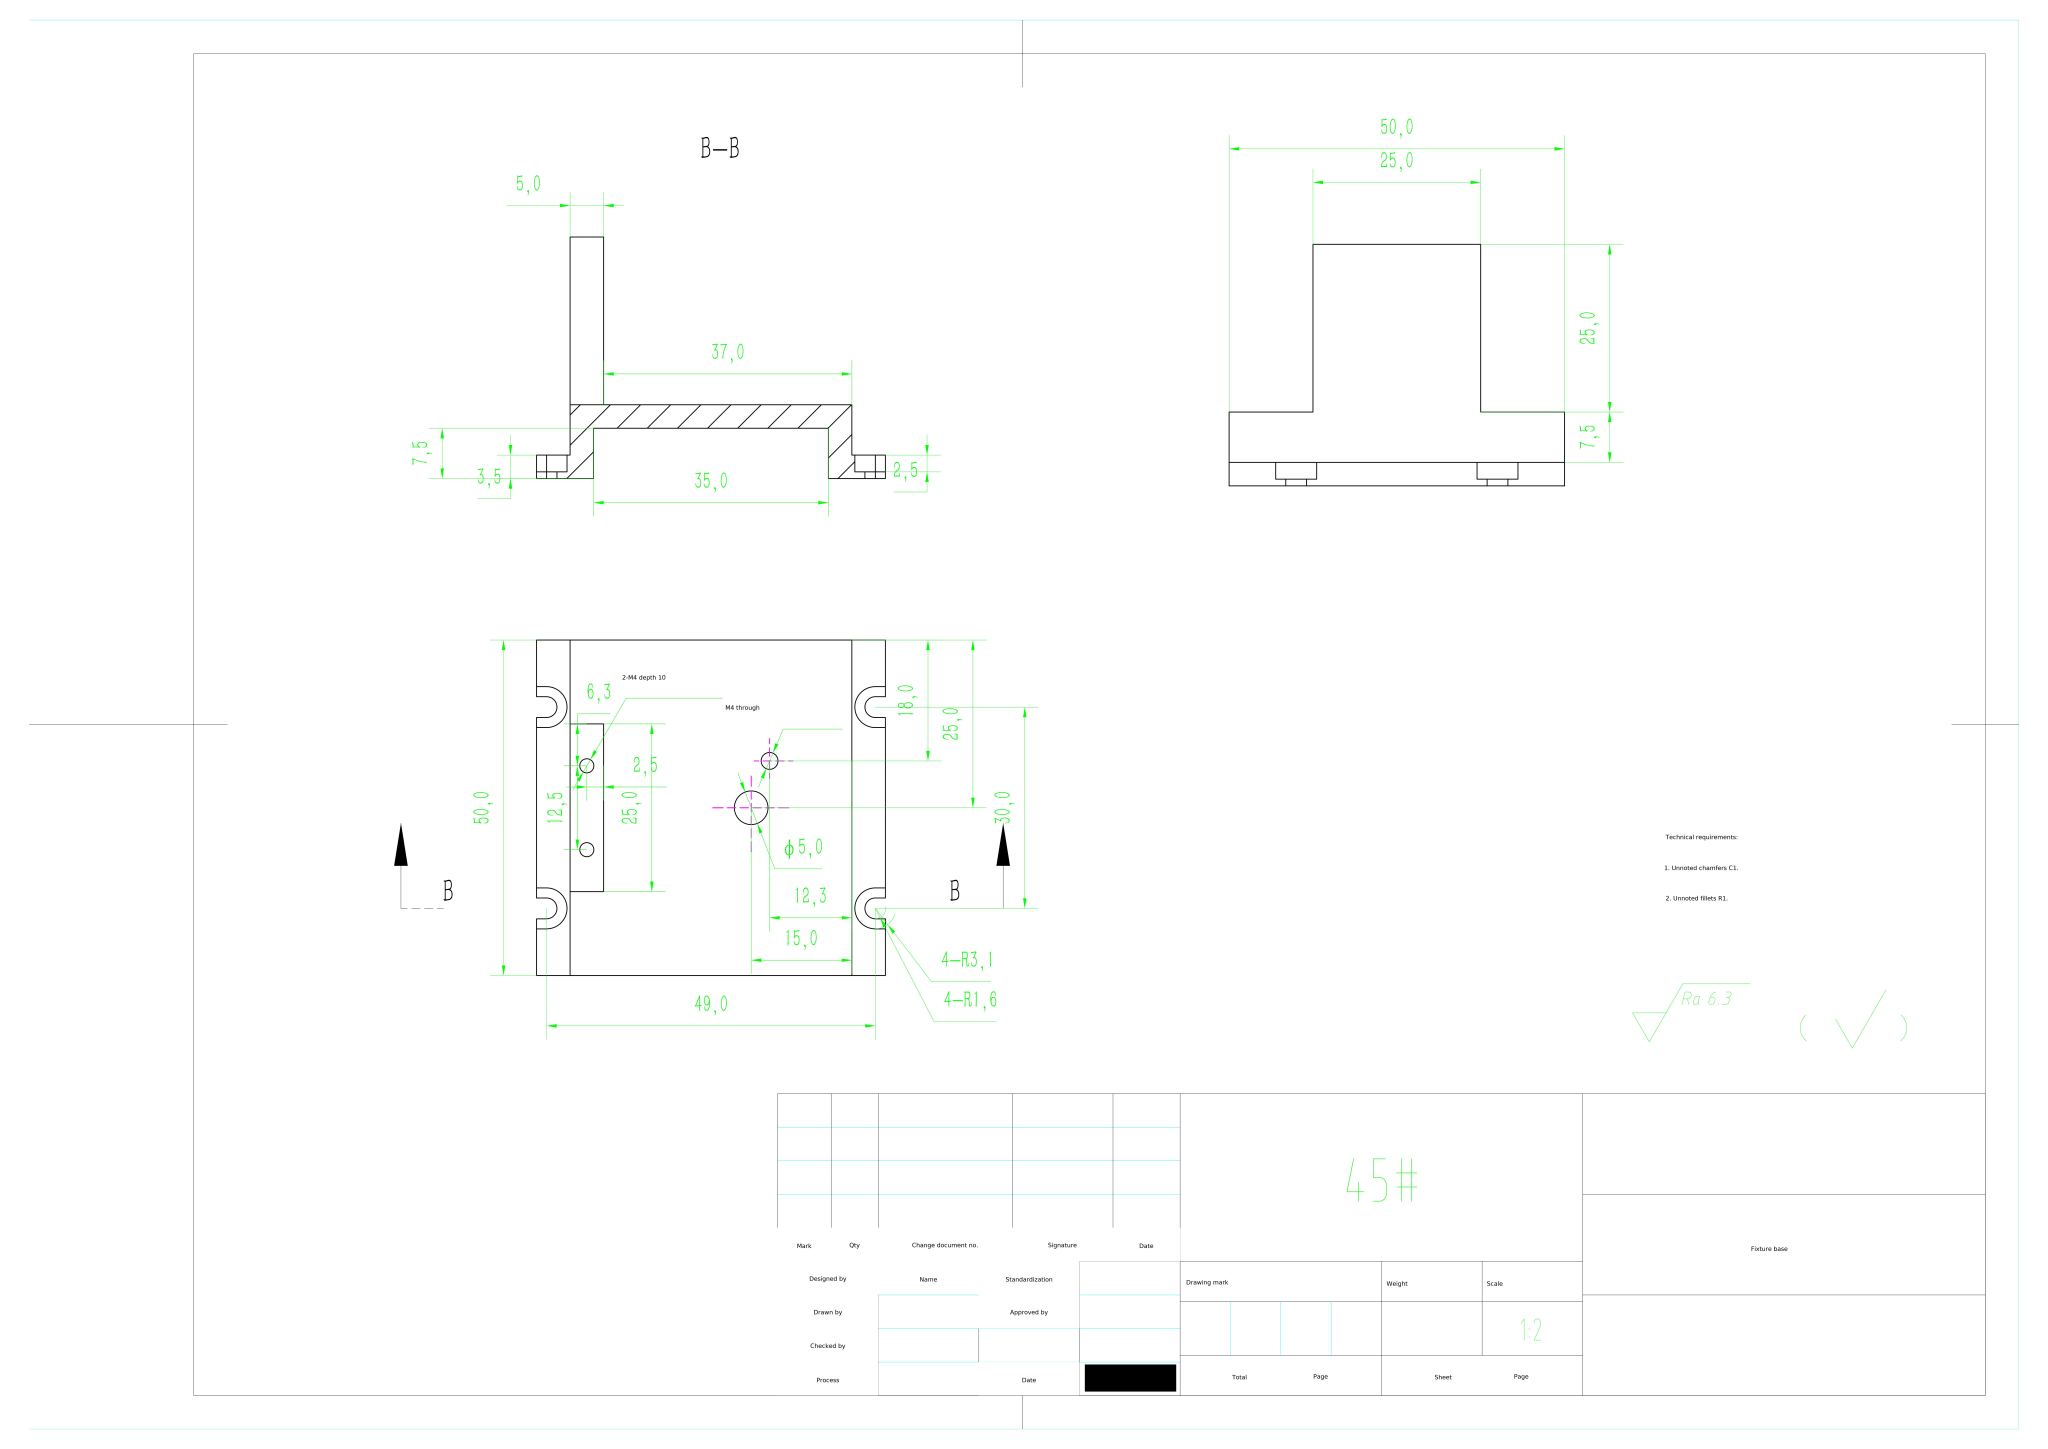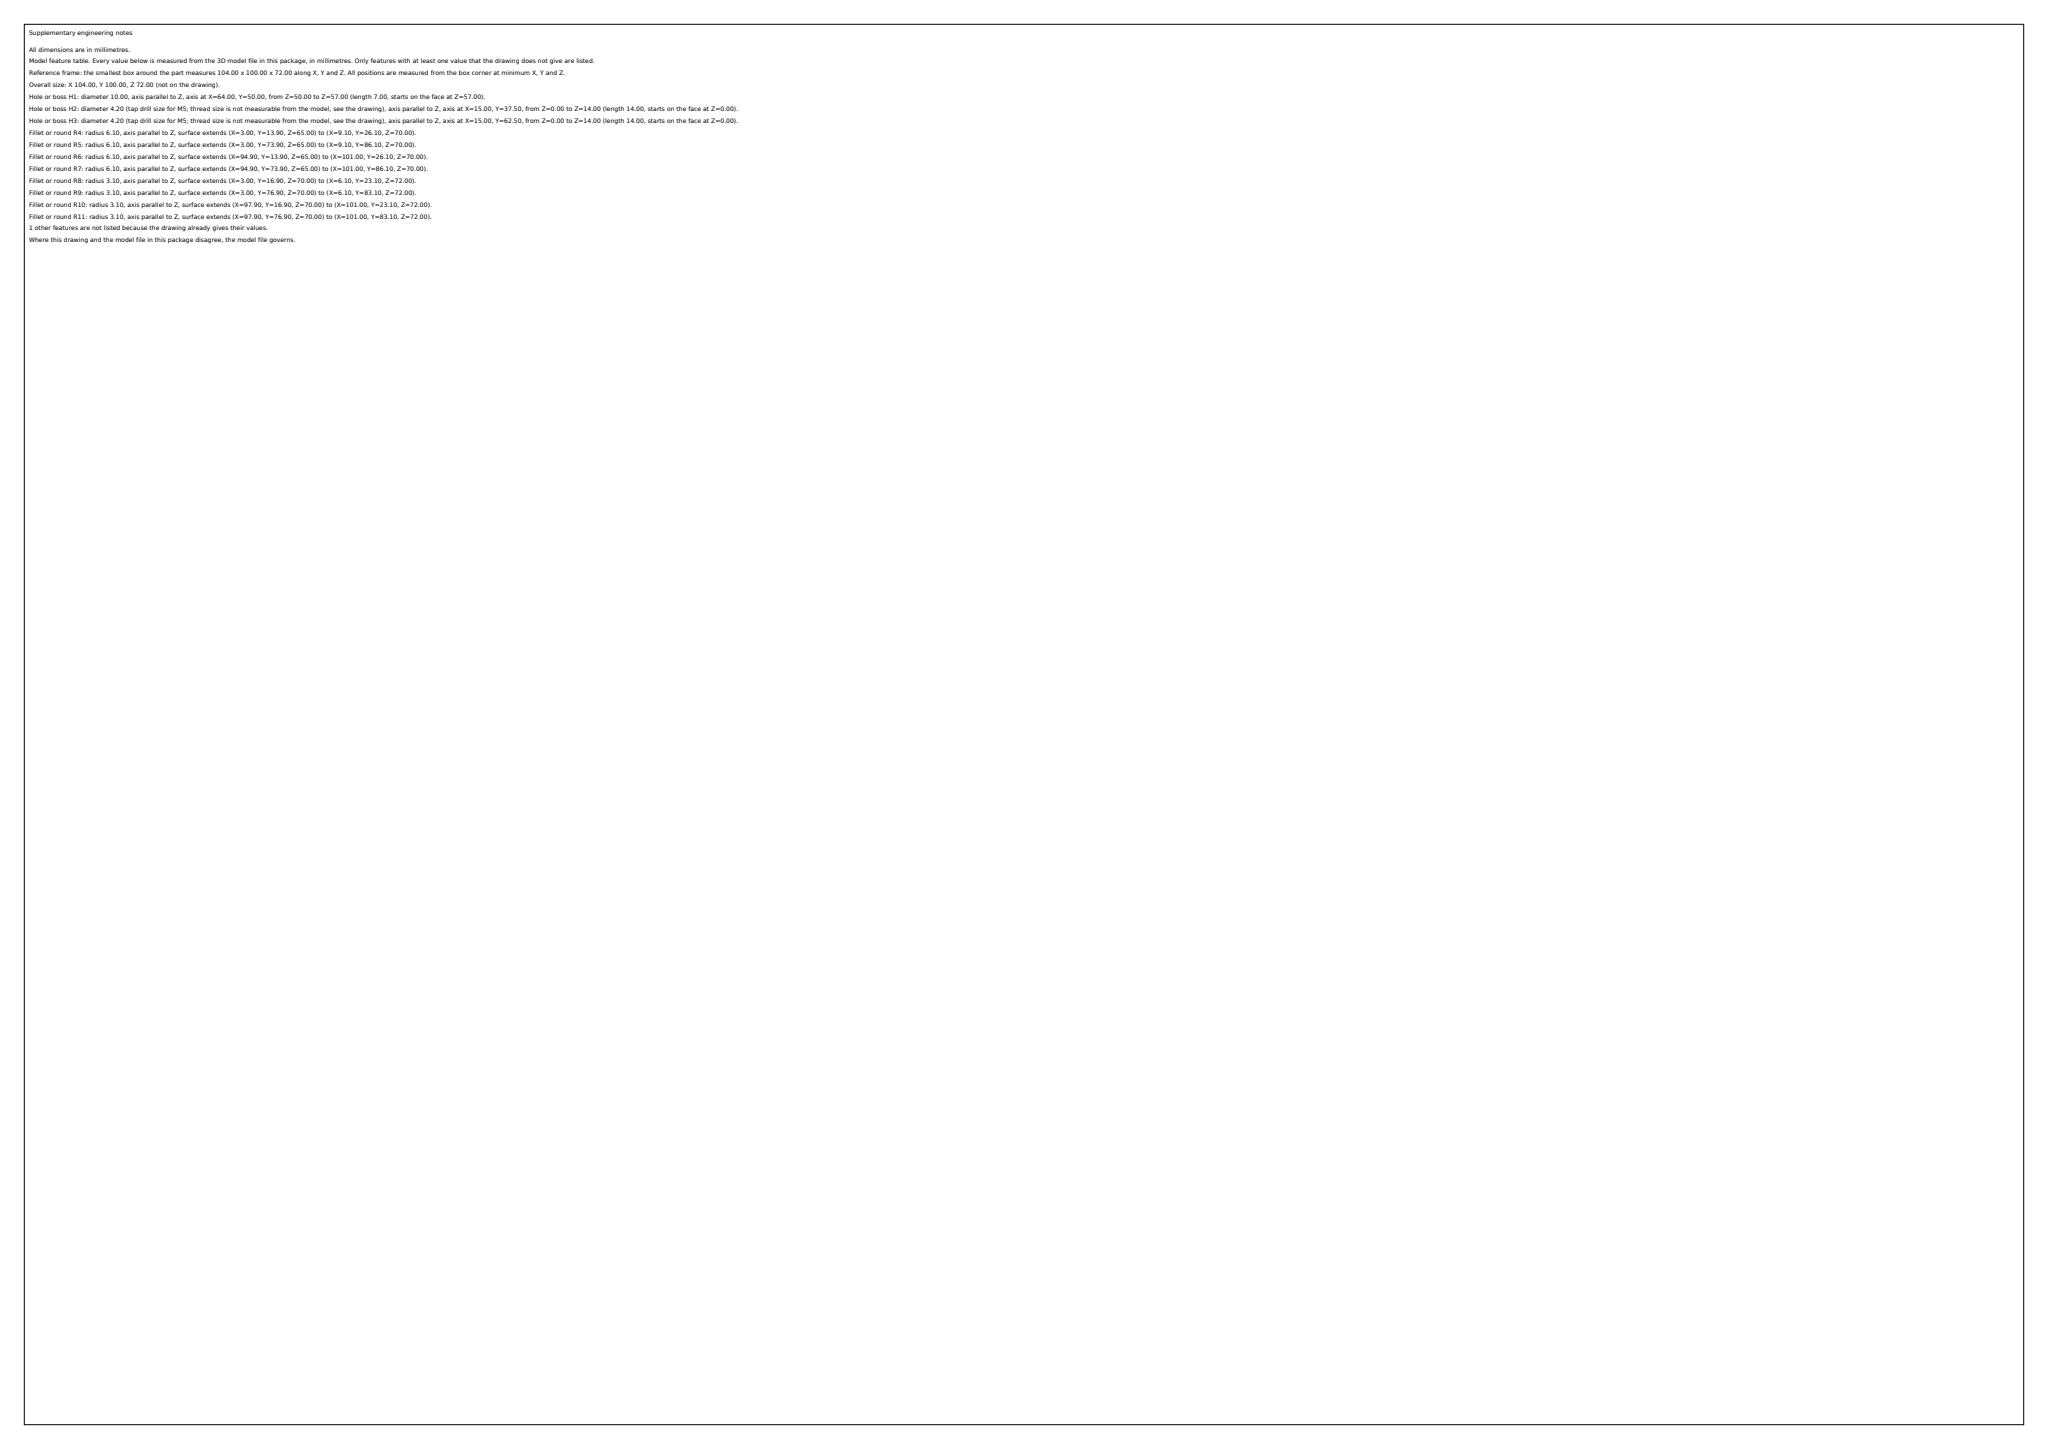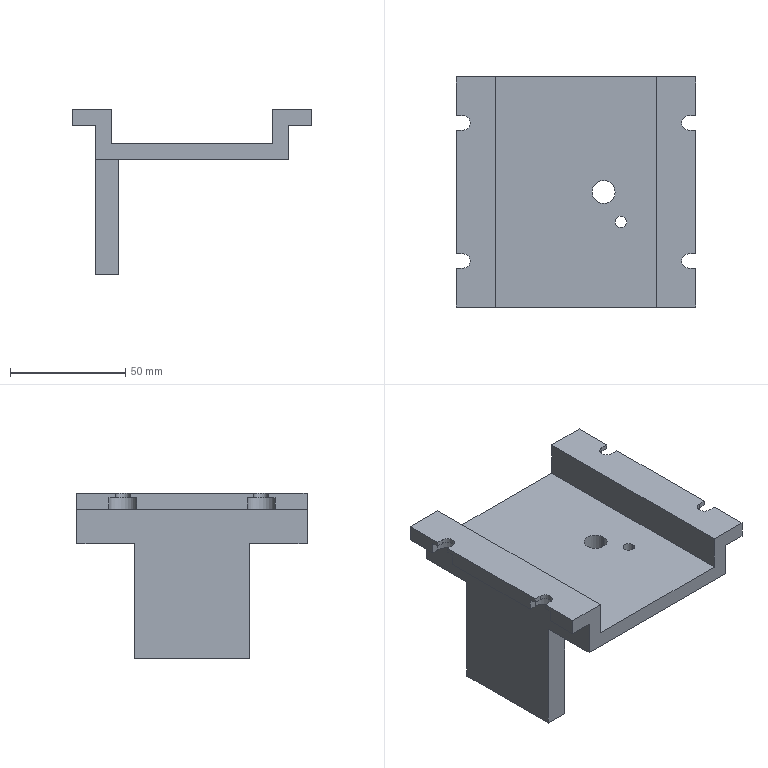Part | SolidWorks | mm | material 45# | 1 solid | 66 faces | box 104 x 100 x 72 mm | volume 115543 mm3 | plane 42 | cylinder 20 | cone 4 | commonest cylinder face diameters 12.2 x6 6.2 x6 4.2 x4 5 x2 10 x2
build123d program:
from build123d import *

# Parameters (mm, degrees)
BOSS_EXTRUDE1_DEPTH   = 100
SKETCH2_W             = 10
SKETCH2_H             = 50
BOSS_EXTRUDE2_DEPTH   = 50
M5_TAPPED_HOLE1_D     = 4.2
M5_TAPPED_HOLE1_DEPTH = 14
M5_TAPPED_HOLE1_TIP   = 1.262
CUT_EXTRUDE1_DEPTH    = 131.111
CUT_EXTRUDE2_DEPTH    = 5
SKETCH7_R             = 5
CUT_EXTRUDE3_DEPTH    = 124.305
M6_TAPPED_HOLE1_D     = 5
M6_TAPPED_HOLE1_DEPTH = 17
M6_TAPPED_HOLE1_TIP   = 1.502


with BuildPart() as part:
    # Sketch1 → Boss-Extrude1 (new body)
    with BuildSketch(Plane(origin=(0, 0, 0), x_dir=(1, 0, 0), z_dir=(0, 1, 0))):
        Polygon((-35, -3.5), (-35, -18.5), (-52, -18.5), (-52, -11.5), (-42, -11.5), (-42, 3.5), (-35, 3.5), (35, 3.5), (42, 3.5), (42, -11.5), (52, -11.5), (52, -18.5), (35, -18.5), (35, -3.5), align=None)
    extrude(amount=BOSS_EXTRUDE1_DEPTH)

    # Sketch2 → Boss-Extrude2 (add)
    with BuildSketch(Plane(origin=(0, 0, -3.5), x_dir=(-1, 0, 0), z_dir=(0, 0, -1))):
        with Locations((37, 50)):
            Rectangle(SKETCH2_W, SKETCH2_H)
    extrude(amount=BOSS_EXTRUDE2_DEPTH)

    # M5 Tapped Hole1
    with Locations(Plane(origin=(0, 0, -53.5), x_dir=(-1, 0, 0), z_dir=(0, 0, -1))):
        with Locations((37, 37.5), (37, 62.5)):
            Hole(M5_TAPPED_HOLE1_D / 2, depth=M5_TAPPED_HOLE1_DEPTH)
            with Locations((0, 0, -(M5_TAPPED_HOLE1_DEPTH + M5_TAPPED_HOLE1_TIP / 2))):  # 118° drill point
                Cone(0, M5_TAPPED_HOLE1_D / 2, M5_TAPPED_HOLE1_TIP, mode=Mode.SUBTRACT)

    # Sketch5 → Cut-Extrude1 (cut, through all)
    with BuildSketch(Plane(origin=(0, 0, 11.5), x_dir=(-1, 0, 0), z_dir=(0, 0, -1))):
        with BuildLine():
            Line((52, 76.9), (49, 76.9))
            ThreePointArc((49, 76.9), (45.9, 80), (49, 83.1))
            Line((49, 83.1), (52, 83.1))
            ThreePointArc((52, 83.1), (55.1, 80), (52, 76.9))
        make_face()
        with BuildLine():
            Line((-52, 83.1), (-49, 83.1))
            ThreePointArc((-49, 83.1), (-45.9, 80), (-49, 76.9))
            Line((-49, 76.9), (-52, 76.9))
            ThreePointArc((-52, 76.9), (-55.1, 80), (-52, 83.1))
        make_face()
        with BuildLine():
            Line((-52, 23.1), (-49, 23.1))
            ThreePointArc((-49, 23.1), (-45.9, 20), (-49, 16.9))
            Line((-49, 16.9), (-52, 16.9))
            ThreePointArc((-52, 16.9), (-55.1, 20), (-52, 23.1))
        make_face()
        with BuildLine():
            Line((52, 16.9), (49, 16.9))
            ThreePointArc((49, 16.9), (45.9, 20), (49, 23.1))
            Line((49, 23.1), (52, 23.1))
            ThreePointArc((52, 23.1), (55.1, 20), (52, 16.9))
        make_face()
    extrude(amount=-CUT_EXTRUDE1_DEPTH, mode=Mode.SUBTRACT)

    # Sketch6 → Cut-Extrude2 (cut)
    with BuildSketch(Plane(origin=(0, 0, 11.5), x_dir=(-1, 0, 0), z_dir=(0, 0, -1))):
        with BuildLine():
            Line((49, 86.1), (60.543, 86.1))
            ThreePointArc((60.543, 86.1), (66.643, 80), (60.543, 73.9))
            Line((60.543, 73.9), (49, 73.9))
            ThreePointArc((49, 73.9), (42.9, 80), (49, 86.1))
        make_face()
        with BuildLine():
            Line((49, 26.1), (61.759, 26.1))
            ThreePointArc((61.759, 26.1), (67.859, 20), (61.759, 13.9))
            Line((61.759, 13.9), (49, 13.9))
            ThreePointArc((49, 13.9), (42.9, 20), (49, 26.1))
        make_face()
        with BuildLine():
            Line((-49, 13.9), (-60.73, 13.9))
            ThreePointArc((-60.73, 13.9), (-66.83, 20), (-60.73, 26.1))
            Line((-60.73, 26.1), (-49, 26.1))
            ThreePointArc((-49, 26.1), (-42.9, 20), (-49, 13.9))
        make_face()
        with BuildLine():
            Line((-49, 73.9), (-62.32, 73.9))
            ThreePointArc((-62.32, 73.9), (-68.42, 80), (-62.32, 86.1))
            Line((-62.32, 86.1), (-49, 86.1))
            ThreePointArc((-49, 86.1), (-42.9, 80), (-49, 73.9))
        make_face()
    extrude(amount=-CUT_EXTRUDE2_DEPTH, mode=Mode.SUBTRACT)

    # Sketch7 → Cut-Extrude3 (cut, through all)
    with BuildSketch(Plane(origin=(0, 0, -3.5), x_dir=(-1, 0, 0), z_dir=(0, 0, -1))):
        with Locations((-12, 50)):
            Circle(SKETCH7_R)
    extrude(amount=-CUT_EXTRUDE3_DEPTH, mode=Mode.SUBTRACT)

    # M6 Tapped Hole1
    with Locations(Plane.XY.offset(3.5)):
        with Locations((19.5, 37.01)):
            Hole(M6_TAPPED_HOLE1_D / 2, depth=M6_TAPPED_HOLE1_DEPTH)
            with Locations((0, 0, -(M6_TAPPED_HOLE1_DEPTH + M6_TAPPED_HOLE1_TIP / 2))):  # 118° drill point
                Cone(0, M6_TAPPED_HOLE1_D / 2, M6_TAPPED_HOLE1_TIP, mode=Mode.SUBTRACT)


solid = part.part